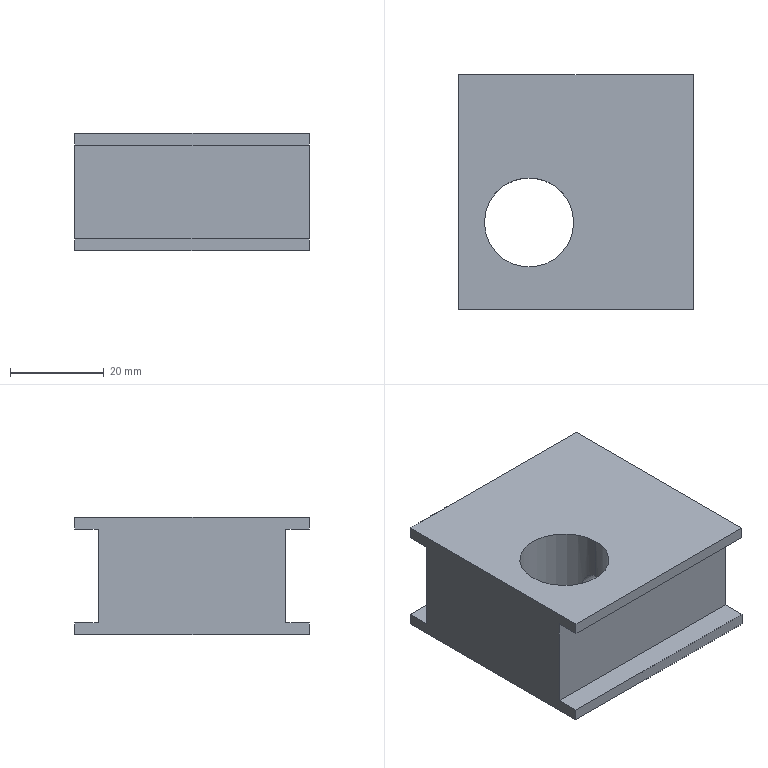Component | SolidWorks | TensionBlock-1 | 1 solid | 18 faces | box 50 x 50 x 25 mm | volume 44480 mm3 | plane 14 | cylinder 4 | commonest cylinder face diameters 6.8 x2 19 x2
build123d program:
from build123d import *

# Parameters (mm, degrees)
SKETCH1_W             = 50
SKETCH1_H             = 50
BOSS_EXTRUDE1_DEPTH   = 12.5
SKETCH2_W             = 20
SKETCH2_H             = 5
CUT_EXTRUDE1_DEPTH    = 58.282
SKETCH3_R             = 9.5
CUT_EXTRUDE2_DEPTH    = 25
M8_TAPPED_HOLE1_D     = 6.8
M8_TAPPED_HOLE1_DEPTH = 35
M8_TAPPED_HOLE1_TIP   = 2.043


with BuildPart() as part:
    # Sketch1 → Boss-Extrude1 (new, symmetric)
    with BuildSketch(Plane(origin=(0, 0, 0), x_dir=(0, 0, -1), z_dir=(1, 0, 0))):
        Rectangle(SKETCH1_W, SKETCH1_H)
    extrude(amount=BOSS_EXTRUDE1_DEPTH, both=True)

    # Sketch2 → Cut-Extrude1 (cut, through all)
    with BuildSketch(Plane(origin=(0, 0, -25), x_dir=(-1, 0, 0), z_dir=(0, 0, -1))):
        with Locations((0, 22.5)):
            Rectangle(SKETCH2_W, SKETCH2_H)
        with Locations((0, -22.5)):
            Rectangle(SKETCH2_W, SKETCH2_H)
    extrude(amount=-CUT_EXTRUDE1_DEPTH, mode=Mode.SUBTRACT)

    # Sketch3 → Cut-Extrude2 (cut)
    with BuildSketch(Plane(origin=(12.5, 0, 0), x_dir=(0, 0, -1), z_dir=(1, 0, 0))):
        with Locations((10, -6.5)):
            Circle(SKETCH3_R)
    extrude(amount=-CUT_EXTRUDE2_DEPTH, mode=Mode.SUBTRACT)

    # M8 Tapped Hole1
    with Locations(Plane.XY.offset(25)):
        with Locations((0, -6.5)):
            Hole(M8_TAPPED_HOLE1_D / 2, depth=M8_TAPPED_HOLE1_DEPTH)
            with Locations((0, 0, -(M8_TAPPED_HOLE1_DEPTH + M8_TAPPED_HOLE1_TIP / 2))):  # 118° drill point
                Cone(0, M8_TAPPED_HOLE1_D / 2, M8_TAPPED_HOLE1_TIP, mode=Mode.SUBTRACT)


solid = part.part

# Placed as in the assembly
solid = solid.moved(Location((235.493, -33.411, 631), (0, 90, 0)))
STEP:
#1=COLOUR_RGB('',0.7922,0.8196,0.9333);
#2=FILL_AREA_STYLE_COLOUR('',#1);
#3=FILL_AREA_STYLE('',(#2));
#4=SURFACE_STYLE_FILL_AREA(#3);
#5=SURFACE_SIDE_STYLE('',(#4));
#6=SURFACE_STYLE_USAGE(.BOTH.,#5);
#7=PRESENTATION_STYLE_ASSIGNMENT((#6));
#8=CARTESIAN_POINT('',(9.252,-1.571,24.976));
#9=VERTEX_POINT('',#8);
#10=CARTESIAN_POINT('',(9.252,-1.571,24.709));
#11=VERTEX_POINT('',#10);
#12=CARTESIAN_POINT('',(9.252,-1.571,24.976));
#13=CARTESIAN_POINT('',(9.252,-1.58,24.976));
#14=CARTESIAN_POINT('',(9.251,-1.589,24.976));
#15=CARTESIAN_POINT('',(9.25,-1.606,24.972));
#16=CARTESIAN_POINT('',(9.249,-1.615,24.969));
#17=CARTESIAN_POINT('',(9.247,-1.631,24.963));
#18=CARTESIAN_POINT('',(9.246,-1.639,24.959));
#19=CARTESIAN_POINT('',(9.243,-1.653,24.949));
#20=CARTESIAN_POINT('',(9.241,-1.66,24.943));
#21=CARTESIAN_POINT('',(9.238,-1.672,24.931));
#22=CARTESIAN_POINT('',(9.236,-1.678,24.924));
#23=CARTESIAN_POINT('',(9.233,-1.687,24.91));
#24=CARTESIAN_POINT('',(9.232,-1.692,24.902));
#25=CARTESIAN_POINT('',(9.23,-1.698,24.886));
#26=CARTESIAN_POINT('',(9.229,-1.701,24.877));
#27=CARTESIAN_POINT('',(9.227,-1.704,24.86));
#28=CARTESIAN_POINT('',(9.227,-1.705,24.851));
#29=CARTESIAN_POINT('',(9.227,-1.705,24.834));
#30=CARTESIAN_POINT('',(9.227,-1.704,24.825));
#31=CARTESIAN_POINT('',(9.229,-1.701,24.808));
#32=CARTESIAN_POINT('',(9.23,-1.698,24.799));
#33=CARTESIAN_POINT('',(9.232,-1.692,24.783));
#34=CARTESIAN_POINT('',(9.233,-1.687,24.775));
#35=CARTESIAN_POINT('',(9.236,-1.678,24.761));
#36=CARTESIAN_POINT('',(9.238,-1.672,24.754));
#37=CARTESIAN_POINT('',(9.241,-1.66,24.742));
#38=CARTESIAN_POINT('',(9.243,-1.653,24.736));
#39=CARTESIAN_POINT('',(9.246,-1.639,24.726));
#40=CARTESIAN_POINT('',(9.247,-1.631,24.722));
#41=CARTESIAN_POINT('',(9.249,-1.615,24.716));
#42=CARTESIAN_POINT('',(9.25,-1.606,24.713));
#43=CARTESIAN_POINT('',(9.251,-1.589,24.71));
#44=CARTESIAN_POINT('',(9.252,-1.58,24.709));
#45=CARTESIAN_POINT('',(9.252,-1.571,24.709));
#46=B_SPLINE_CURVE_WITH_KNOTS('',3,(#12,#13,#14,#15,#16,#17,#18,#19,#20,#21,#22,#23,#24,#25,#26,#27,#28,#29,#30,#31,#32,#33,#34,#35,#36,#37,#38,#39,#40,#41,#42,#43,#44,#45),.UNSPECIFIED.,.F.,.F.,(4,2,2,2,2,2,2,2,2,2,2,2,2,2,2,2,4),(0.01072,0.01139,0.01206,0.01273,0.0134,0.01407,0.01474,0.01541,0.01608,0.01675,0.01742,0.01809,0.01876,0.01943,0.0201,0.02077,0.02144),.UNSPECIFIED.);
#47=EDGE_CURVE('',#9,#11,#46,.T.);
#48=ORIENTED_EDGE('',*,*,#47,.F.);
#49=CARTESIAN_POINT('',(10.256,-1.571,24.976));
#50=VERTEX_POINT('',#49);
#51=CARTESIAN_POINT('',(10.256,-1.571,24.976));
#52=DIRECTION('',(1.,-0.,0.));
#53=VECTOR('',#52,39.37);
#54=LINE('',#51,#53);
#55=EDGE_CURVE('',#9,#50,#54,.T.);
#56=ORIENTED_EDGE('',*,*,#55,.T.);
#57=CARTESIAN_POINT('',(10.256,-1.571,24.709));
#58=VERTEX_POINT('',#57);
#59=CARTESIAN_POINT('',(10.256,-1.571,24.843));
#60=DIRECTION('',(1.,-0.,0.));
#61=DIRECTION('',(0.,0.,-1.));
#62=AXIS2_PLACEMENT_3D('',#59,#60,#61);
#63=CIRCLE('',#62,0.1339);
#64=EDGE_CURVE('',#50,#58,#63,.T.);
#65=ORIENTED_EDGE('',*,*,#64,.T.);
#66=CARTESIAN_POINT('',(10.256,-1.571,24.709));
#67=DIRECTION('',(1.,-0.,0.));
#68=VECTOR('',#67,39.37);
#69=LINE('',#66,#68);
#70=EDGE_CURVE('',#11,#58,#69,.T.);
#71=ORIENTED_EDGE('',*,*,#70,.F.);
#72=EDGE_LOOP('',(#48,#56,#65,#71));
#73=FACE_OUTER_BOUND('',#72,.T.);
#74=CARTESIAN_POINT('',(10.256,-1.571,24.843));
#75=DIRECTION('',(1.,-0.,0.));
#76=DIRECTION('',(0.,0.,-1.));
#77=AXIS2_PLACEMENT_3D('',#74,#75,#76);
#78=CYLINDRICAL_SURFACE('',#77,0.1339);
#79=ADVANCED_FACE('',(#73),#78,.F.);
#80=CARTESIAN_POINT('',(9.252,-1.571,25.335));
#81=VERTEX_POINT('',#80);
#82=CARTESIAN_POINT('',(8.504,-1.571,25.335));
#83=VERTEX_POINT('',#82);
#84=CARTESIAN_POINT('',(8.878,-1.571,25.335));
#85=DIRECTION('',(0.,0.,-1.));
#86=DIRECTION('',(-1.,0.,0.));
#87=AXIS2_PLACEMENT_3D('',#84,#85,#86);
#88=CIRCLE('',#87,0.374);
#89=EDGE_CURVE('',#81,#83,#88,.T.);
#90=ORIENTED_EDGE('',*,*,#89,.F.);
#91=CARTESIAN_POINT('',(9.252,-1.571,25.335));
#92=DIRECTION('',(0.,0.,-1.));
#93=VECTOR('',#92,39.37);
#94=LINE('',#91,#93);
#95=EDGE_CURVE('',#81,#9,#94,.T.);
#96=ORIENTED_EDGE('',*,*,#95,.T.);
#97=ORIENTED_EDGE('',*,*,#47,.T.);
#98=CARTESIAN_POINT('',(9.252,-1.571,24.35));
#99=VERTEX_POINT('',#98);
#100=CARTESIAN_POINT('',(9.252,-1.571,25.335));
#101=DIRECTION('',(0.,0.,-1.));
#102=VECTOR('',#101,39.37);
#103=LINE('',#100,#102);
#104=EDGE_CURVE('',#11,#99,#103,.T.);
#105=ORIENTED_EDGE('',*,*,#104,.T.);
#106=CARTESIAN_POINT('',(8.504,-1.571,24.35));
#107=VERTEX_POINT('',#106);
#108=CARTESIAN_POINT('',(8.878,-1.571,24.35));
#109=DIRECTION('',(0.,0.,-1.));
#110=DIRECTION('',(-1.,0.,0.));
#111=AXIS2_PLACEMENT_3D('',#108,#109,#110);
#112=CIRCLE('',#111,0.374);
#113=EDGE_CURVE('',#99,#107,#112,.T.);
#114=ORIENTED_EDGE('',*,*,#113,.T.);
#115=CARTESIAN_POINT('',(8.504,-1.571,25.335));
#116=DIRECTION('',(0.,0.,-1.));
#117=VECTOR('',#116,39.37);
#118=LINE('',#115,#117);
#119=EDGE_CURVE('',#83,#107,#118,.T.);
#120=ORIENTED_EDGE('',*,*,#119,.F.);
#121=EDGE_LOOP('',(#90,#96,#97,#105,#114,#120));
#122=FACE_OUTER_BOUND('',#121,.T.);
#123=CARTESIAN_POINT('',(8.878,-1.571,25.335));
#124=DIRECTION('',(0.,0.,-1.));
#125=DIRECTION('',(-1.,0.,0.));
#126=AXIS2_PLACEMENT_3D('',#123,#124,#125);
#127=CYLINDRICAL_SURFACE('',#126,0.374);
#128=ADVANCED_FACE('',(#122),#127,.F.);
#129=CARTESIAN_POINT('',(10.256,-2.3,24.35));
#130=VERTEX_POINT('',#129);
#131=CARTESIAN_POINT('',(10.256,-2.3,24.449));
#132=VERTEX_POINT('',#131);
#133=CARTESIAN_POINT('',(10.256,-2.3,24.35));
#134=DIRECTION('',(-0.,-0.,1.));
#135=VECTOR('',#134,39.37);
#136=LINE('',#133,#135);
#137=EDGE_CURVE('',#130,#132,#136,.T.);
#138=ORIENTED_EDGE('',*,*,#137,.T.);
#139=CARTESIAN_POINT('',(8.287,-2.3,24.449));
#140=VERTEX_POINT('',#139);
#141=CARTESIAN_POINT('',(10.256,-2.3,24.449));
#142=DIRECTION('',(-1.,0.,-0.));
#143=VECTOR('',#142,39.37);
#144=LINE('',#141,#143);
#145=EDGE_CURVE('',#132,#140,#144,.T.);
#146=ORIENTED_EDGE('',*,*,#145,.T.);
#147=CARTESIAN_POINT('',(8.287,-2.3,24.35));
#148=VERTEX_POINT('',#147);
#149=CARTESIAN_POINT('',(8.287,-2.3,24.35));
#150=DIRECTION('',(-0.,-0.,1.));
#151=VECTOR('',#150,39.37);
#152=LINE('',#149,#151);
#153=EDGE_CURVE('',#148,#140,#152,.T.);
#154=ORIENTED_EDGE('',*,*,#153,.F.);
#155=CARTESIAN_POINT('',(8.287,-2.3,24.35));
#156=DIRECTION('',(-1.,0.,-0.));
#157=VECTOR('',#156,39.37);
#158=LINE('',#155,#157);
#159=EDGE_CURVE('',#130,#148,#158,.T.);
#160=ORIENTED_EDGE('',*,*,#159,.F.);
#161=EDGE_LOOP('',(#138,#146,#154,#160));
#162=FACE_OUTER_BOUND('',#161,.T.);
#163=CARTESIAN_POINT('',(8.287,-2.3,24.35));
#164=DIRECTION('',(0.,1.,0.));
#165=DIRECTION('',(1.,-0.,0.));
#166=AXIS2_PLACEMENT_3D('',#163,#164,#165);
#167=PLANE('',#166);
#168=ADVANCED_FACE('',(#162),#167,.F.);
#169=CARTESIAN_POINT('',(8.287,-0.3312,24.35));
#170=VERTEX_POINT('',#169);
#171=CARTESIAN_POINT('',(8.287,-0.3312,24.449));
#172=VERTEX_POINT('',#171);
#173=CARTESIAN_POINT('',(8.287,-0.3312,24.35));
#174=DIRECTION('',(-0.,-0.,1.));
#175=VECTOR('',#174,39.37);
#176=LINE('',#173,#175);
#177=EDGE_CURVE('',#170,#172,#176,.T.);
#178=ORIENTED_EDGE('',*,*,#177,.T.);
#179=CARTESIAN_POINT('',(10.256,-0.3312,24.449));
#180=VERTEX_POINT('',#179);
#181=CARTESIAN_POINT('',(10.256,-0.3312,24.449));
#182=DIRECTION('',(-1.,0.,-0.));
#183=VECTOR('',#182,39.37);
#184=LINE('',#181,#183);
#185=EDGE_CURVE('',#180,#172,#184,.T.);
#186=ORIENTED_EDGE('',*,*,#185,.F.);
#187=CARTESIAN_POINT('',(10.256,-0.3312,24.35));
#188=VERTEX_POINT('',#187);
#189=CARTESIAN_POINT('',(10.256,-0.3312,24.35));
#190=DIRECTION('',(-0.,-0.,1.));
#191=VECTOR('',#190,39.37);
#192=LINE('',#189,#191);
#193=EDGE_CURVE('',#188,#180,#192,.T.);
#194=ORIENTED_EDGE('',*,*,#193,.F.);
#195=CARTESIAN_POINT('',(8.287,-0.3312,24.35));
#196=DIRECTION('',(1.,-0.,0.));
#197=VECTOR('',#196,39.37);
#198=LINE('',#195,#197);
#199=EDGE_CURVE('',#170,#188,#198,.T.);
#200=ORIENTED_EDGE('',*,*,#199,.F.);
#201=EDGE_LOOP('',(#178,#186,#194,#200));
#202=FACE_OUTER_BOUND('',#201,.T.);
#203=CARTESIAN_POINT('',(8.287,-0.3312,24.35));
#204=DIRECTION('',(-0.,-1.,-0.));
#205=DIRECTION('',(-1.,0.,-0.));
#206=AXIS2_PLACEMENT_3D('',#203,#204,#205);
#207=PLANE('',#206);
#208=ADVANCED_FACE('',(#202),#207,.F.);
#209=CARTESIAN_POINT('',(10.256,-1.571,24.843));
#210=DIRECTION('',(1.,-0.,0.));
#211=DIRECTION('',(0.,0.,-1.));
#212=AXIS2_PLACEMENT_3D('',#209,#210,#211);
#213=CIRCLE('',#212,0.1339);
#214=EDGE_CURVE('',#58,#50,#213,.T.);
#215=ORIENTED_EDGE('',*,*,#214,.F.);
#216=ORIENTED_EDGE('',*,*,#64,.F.);
#217=EDGE_LOOP('',(#215,#216));
#218=FACE_BOUND('',#217,.T.);
#219=CARTESIAN_POINT('',(10.256,-2.103,25.236));
#220=VERTEX_POINT('',#219);
#221=CARTESIAN_POINT('',(10.256,-2.103,24.449));
#222=VERTEX_POINT('',#221);
#223=CARTESIAN_POINT('',(10.256,-2.103,24.449));
#224=DIRECTION('',(0.,0.,-1.));
#225=VECTOR('',#224,39.37);
#226=LINE('',#223,#225);
#227=EDGE_CURVE('',#220,#222,#226,.T.);
#228=ORIENTED_EDGE('',*,*,#227,.T.);
#229=CARTESIAN_POINT('',(10.256,-2.3,24.449));
#230=DIRECTION('',(-0.,-1.,-0.));
#231=VECTOR('',#230,39.37);
#232=LINE('',#229,#231);
#233=EDGE_CURVE('',#222,#132,#232,.T.);
#234=ORIENTED_EDGE('',*,*,#233,.T.);
#235=ORIENTED_EDGE('',*,*,#137,.F.);
#236=CARTESIAN_POINT('',(10.256,-2.3,24.35));
#237=DIRECTION('',(-0.,-1.,-0.));
#238=VECTOR('',#237,39.37);
#239=LINE('',#236,#238);
#240=EDGE_CURVE('',#188,#130,#239,.T.);
#241=ORIENTED_EDGE('',*,*,#240,.F.);
#242=ORIENTED_EDGE('',*,*,#193,.T.);
#243=CARTESIAN_POINT('',(10.256,-0.528,24.449));
#244=VERTEX_POINT('',#243);
#245=CARTESIAN_POINT('',(10.256,-0.3312,24.449));
#246=DIRECTION('',(-0.,-1.,0.));
#247=VECTOR('',#246,39.37);
#248=LINE('',#245,#247);
#249=EDGE_CURVE('',#180,#244,#248,.T.);
#250=ORIENTED_EDGE('',*,*,#249,.T.);
#251=CARTESIAN_POINT('',(10.256,-0.528,25.236));
#252=VERTEX_POINT('',#251);
#253=CARTESIAN_POINT('',(10.256,-0.528,24.449));
#254=DIRECTION('',(-0.,-0.,1.));
#255=VECTOR('',#254,39.37);
#256=LINE('',#253,#255);
#257=EDGE_CURVE('',#244,#252,#256,.T.);
#258=ORIENTED_EDGE('',*,*,#257,.T.);
#259=CARTESIAN_POINT('',(10.256,-0.3312,25.236));
#260=VERTEX_POINT('',#259);
#261=CARTESIAN_POINT('',(10.256,-0.3312,25.236));
#262=DIRECTION('',(0.,1.,0.));
#263=VECTOR('',#262,39.37);
#264=LINE('',#261,#263);
#265=EDGE_CURVE('',#252,#260,#264,.T.);
#266=ORIENTED_EDGE('',*,*,#265,.T.);
#267=CARTESIAN_POINT('',(10.256,-0.3312,25.335));
#268=VERTEX_POINT('',#267);
#269=CARTESIAN_POINT('',(10.256,-0.3312,24.35));
#270=DIRECTION('',(-0.,-0.,1.));
#271=VECTOR('',#270,39.37);
#272=LINE('',#269,#271);
#273=EDGE_CURVE('',#260,#268,#272,.T.);
#274=ORIENTED_EDGE('',*,*,#273,.T.);
#275=CARTESIAN_POINT('',(10.256,-2.3,25.335));
#276=VERTEX_POINT('',#275);
#277=CARTESIAN_POINT('',(10.256,-2.3,25.335));
#278=DIRECTION('',(-0.,-1.,-0.));
#279=VECTOR('',#278,39.37);
#280=LINE('',#277,#279);
#281=EDGE_CURVE('',#268,#276,#280,.T.);
#282=ORIENTED_EDGE('',*,*,#281,.T.);
#283=CARTESIAN_POINT('',(10.256,-2.3,25.236));
#284=VERTEX_POINT('',#283);
#285=CARTESIAN_POINT('',(10.256,-2.3,24.35));
#286=DIRECTION('',(-0.,-0.,1.));
#287=VECTOR('',#286,39.37);
#288=LINE('',#285,#287);
#289=EDGE_CURVE('',#284,#276,#288,.T.);
#290=ORIENTED_EDGE('',*,*,#289,.F.);
#291=CARTESIAN_POINT('',(10.256,-2.3,25.236));
#292=DIRECTION('',(0.,1.,0.));
#293=VECTOR('',#292,39.37);
#294=LINE('',#291,#293);
#295=EDGE_CURVE('',#284,#220,#294,.T.);
#296=ORIENTED_EDGE('',*,*,#295,.T.);
#297=EDGE_LOOP('',(#228,#234,#235,#241,#242,#250,#258,#266,#274,#282,#290,#296));
#298=FACE_OUTER_BOUND('',#297,.T.);
#299=CARTESIAN_POINT('',(10.256,-2.3,24.35));
#300=DIRECTION('',(-1.,0.,-0.));
#301=DIRECTION('',(-0.,-0.,1.));
#302=AXIS2_PLACEMENT_3D('',#299,#300,#301);
#303=PLANE('',#302);
#304=ADVANCED_FACE('',(#218,#298),#303,.F.);
#305=CARTESIAN_POINT('',(8.287,-2.3,25.236));
#306=VERTEX_POINT('',#305);
#307=CARTESIAN_POINT('',(8.287,-2.3,25.335));
#308=VERTEX_POINT('',#307);
#309=CARTESIAN_POINT('',(8.287,-2.3,24.35));
#310=DIRECTION('',(-0.,-0.,1.));
#311=VECTOR('',#310,39.37);
#312=LINE('',#309,#311);
#313=EDGE_CURVE('',#306,#308,#312,.T.);
#314=ORIENTED_EDGE('',*,*,#313,.F.);
#315=CARTESIAN_POINT('',(10.256,-2.3,25.236));
#316=DIRECTION('',(-1.,0.,-0.));
#317=VECTOR('',#316,39.37);
#318=LINE('',#315,#317);
#319=EDGE_CURVE('',#284,#306,#318,.T.);
#320=ORIENTED_EDGE('',*,*,#319,.F.);
#321=ORIENTED_EDGE('',*,*,#289,.T.);
#322=CARTESIAN_POINT('',(8.287,-2.3,25.335));
#323=DIRECTION('',(-1.,0.,-0.));
#324=VECTOR('',#323,39.37);
#325=LINE('',#322,#324);
#326=EDGE_CURVE('',#276,#308,#325,.T.);
#327=ORIENTED_EDGE('',*,*,#326,.T.);
#328=EDGE_LOOP('',(#314,#320,#321,#327));
#329=FACE_OUTER_BOUND('',#328,.T.);
#330=CARTESIAN_POINT('',(8.287,-2.3,24.35));
#331=DIRECTION('',(0.,1.,0.));
#332=DIRECTION('',(1.,-0.,0.));
#333=AXIS2_PLACEMENT_3D('',#330,#331,#332);
#334=PLANE('',#333);
#335=ADVANCED_FACE('',(#329),#334,.F.);
#336=ORIENTED_EDGE('',*,*,#153,.T.);
#337=CARTESIAN_POINT('',(8.287,-2.103,24.449));
#338=VERTEX_POINT('',#337);
#339=CARTESIAN_POINT('',(8.287,-2.3,24.449));
#340=DIRECTION('',(-0.,-1.,-0.));
#341=VECTOR('',#340,39.37);
#342=LINE('',#339,#341);
#343=EDGE_CURVE('',#338,#140,#342,.T.);
#344=ORIENTED_EDGE('',*,*,#343,.F.);
#345=CARTESIAN_POINT('',(8.287,-2.103,25.236));
#346=VERTEX_POINT('',#345);
#347=CARTESIAN_POINT('',(8.287,-2.103,24.449));
#348=DIRECTION('',(0.,0.,-1.));
#349=VECTOR('',#348,39.37);
#350=LINE('',#347,#349);
#351=EDGE_CURVE('',#346,#338,#350,.T.);
#352=ORIENTED_EDGE('',*,*,#351,.F.);
#353=CARTESIAN_POINT('',(8.287,-2.3,25.236));
#354=DIRECTION('',(0.,1.,0.));
#355=VECTOR('',#354,39.37);
#356=LINE('',#353,#355);
#357=EDGE_CURVE('',#306,#346,#356,.T.);
#358=ORIENTED_EDGE('',*,*,#357,.F.);
#359=ORIENTED_EDGE('',*,*,#313,.T.);
#360=CARTESIAN_POINT('',(8.287,-0.3312,25.335));
#361=VERTEX_POINT('',#360);
#362=CARTESIAN_POINT('',(8.287,-2.3,25.335));
#363=DIRECTION('',(0.,1.,0.));
#364=VECTOR('',#363,39.37);
#365=LINE('',#362,#364);
#366=EDGE_CURVE('',#308,#361,#365,.T.);
#367=ORIENTED_EDGE('',*,*,#366,.T.);
#368=CARTESIAN_POINT('',(8.287,-0.3312,25.236));
#369=VERTEX_POINT('',#368);
#370=CARTESIAN_POINT('',(8.287,-0.3312,24.35));
#371=DIRECTION('',(-0.,-0.,1.));
#372=VECTOR('',#371,39.37);
#373=LINE('',#370,#372);
#374=EDGE_CURVE('',#369,#361,#373,.T.);
#375=ORIENTED_EDGE('',*,*,#374,.F.);
#376=CARTESIAN_POINT('',(8.287,-0.528,25.236));
#377=VERTEX_POINT('',#376);
#378=CARTESIAN_POINT('',(8.287,-0.3312,25.236));
#379=DIRECTION('',(0.,1.,0.));
#380=VECTOR('',#379,39.37);
#381=LINE('',#378,#380);
#382=EDGE_CURVE('',#377,#369,#381,.T.);
#383=ORIENTED_EDGE('',*,*,#382,.F.);
#384=CARTESIAN_POINT('',(8.287,-0.528,24.449));
#385=VERTEX_POINT('',#384);
#386=CARTESIAN_POINT('',(8.287,-0.528,24.449));
#387=DIRECTION('',(-0.,-0.,1.));
#388=VECTOR('',#387,39.37);
#389=LINE('',#386,#388);
#390=EDGE_CURVE('',#385,#377,#389,.T.);
#391=ORIENTED_EDGE('',*,*,#390,.F.);
#392=CARTESIAN_POINT('',(8.287,-0.3312,24.449));
#393=DIRECTION('',(-0.,-1.,0.));
#394=VECTOR('',#393,39.37);
#395=LINE('',#392,#394);
#396=EDGE_CURVE('',#172,#385,#395,.T.);
#397=ORIENTED_EDGE('',*,*,#396,.F.);
#398=ORIENTED_EDGE('',*,*,#177,.F.);
#399=CARTESIAN_POINT('',(8.287,-2.3,24.35));
#400=DIRECTION('',(0.,1.,0.));
#401=VECTOR('',#400,39.37);
#402=LINE('',#399,#401);
#403=EDGE_CURVE('',#148,#170,#402,.T.);
#404=ORIENTED_EDGE('',*,*,#403,.F.);
#405=EDGE_LOOP('',(#336,#344,#352,#358,#359,#367,#375,#383,#391,#397,#398,#404));
#406=FACE_OUTER_BOUND('',#405,.T.);
#407=CARTESIAN_POINT('',(8.287,-2.3,24.35));
#408=DIRECTION('',(1.,-0.,0.));
#409=DIRECTION('',(0.,0.,-1.));
#410=AXIS2_PLACEMENT_3D('',#407,#408,#409);
#411=PLANE('',#410);
#412=ADVANCED_FACE('',(#406),#411,.F.);
#413=ORIENTED_EDGE('',*,*,#273,.F.);
#414=CARTESIAN_POINT('',(10.256,-0.3312,25.236));
#415=DIRECTION('',(-1.,0.,-0.));
#416=VECTOR('',#415,39.37);
#417=LINE('',#414,#416);
#418=EDGE_CURVE('',#260,#369,#417,.T.);
#419=ORIENTED_EDGE('',*,*,#418,.T.);
#420=ORIENTED_EDGE('',*,*,#374,.T.);
#421=CARTESIAN_POINT('',(8.287,-0.3312,25.335));
#422=DIRECTION('',(1.,-0.,0.));
#423=VECTOR('',#422,39.37);
#424=LINE('',#421,#423);
#425=EDGE_CURVE('',#361,#268,#424,.T.);
#426=ORIENTED_EDGE('',*,*,#425,.T.);
#427=EDGE_LOOP('',(#413,#419,#420,#426));
#428=FACE_OUTER_BOUND('',#427,.T.);
#429=CARTESIAN_POINT('',(8.287,-0.3312,24.35));
#430=DIRECTION('',(-0.,-1.,-0.));
#431=DIRECTION('',(-1.,0.,-0.));
#432=AXIS2_PLACEMENT_3D('',#429,#430,#431);
#433=PLANE('',#432);
#434=ADVANCED_FACE('',(#428),#433,.F.);
#435=CARTESIAN_POINT('',(8.878,-1.571,24.35));
#436=DIRECTION('',(0.,0.,-1.));
#437=DIRECTION('',(-1.,0.,0.));
#438=AXIS2_PLACEMENT_3D('',#435,#436,#437);
#439=CIRCLE('',#438,0.374);
#440=EDGE_CURVE('',#107,#99,#439,.T.);
#441=ORIENTED_EDGE('',*,*,#440,.F.);
#442=ORIENTED_EDGE('',*,*,#113,.F.);
#443=EDGE_LOOP('',(#441,#442));
#444=FACE_BOUND('',#443,.T.);
#445=ORIENTED_EDGE('',*,*,#240,.T.);
#446=ORIENTED_EDGE('',*,*,#159,.T.);
#447=ORIENTED_EDGE('',*,*,#403,.T.);
#448=ORIENTED_EDGE('',*,*,#199,.T.);
#449=EDGE_LOOP('',(#445,#446,#447,#448));
#450=FACE_OUTER_BOUND('',#449,.T.);
#451=CARTESIAN_POINT('',(9.271,-1.315,24.35));
#452=DIRECTION('',(0.,0.,-1.));
#453=DIRECTION('',(-1.,0.,-0.));
#454=AXIS2_PLACEMENT_3D('',#451,#452,#453);
#455=PLANE('',#454);
#456=ADVANCED_FACE('',(#444,#450),#455,.T.);
#457=CARTESIAN_POINT('',(8.878,-1.571,25.335));
#458=DIRECTION('',(0.,0.,-1.));
#459=DIRECTION('',(-1.,0.,0.));
#460=AXIS2_PLACEMENT_3D('',#457,#458,#459);
#461=CIRCLE('',#460,0.374);
#462=EDGE_CURVE('',#83,#81,#461,.T.);
#463=ORIENTED_EDGE('',*,*,#462,.T.);
#464=ORIENTED_EDGE('',*,*,#89,.T.);
#465=EDGE_LOOP('',(#463,#464));
#466=FACE_BOUND('',#465,.T.);
#467=ORIENTED_EDGE('',*,*,#281,.F.);
#468=ORIENTED_EDGE('',*,*,#425,.F.);
#469=ORIENTED_EDGE('',*,*,#366,.F.);
#470=ORIENTED_EDGE('',*,*,#326,.F.);
#471=EDGE_LOOP('',(#467,#468,#469,#470));
#472=FACE_OUTER_BOUND('',#471,.T.);
#473=CARTESIAN_POINT('',(9.271,-1.315,25.335));
#474=DIRECTION('',(0.,0.,-1.));
#475=DIRECTION('',(-1.,0.,-0.));
#476=AXIS2_PLACEMENT_3D('',#473,#474,#475);
#477=PLANE('',#476);
#478=ADVANCED_FACE('',(#466,#472),#477,.F.);
#479=ORIENTED_EDGE('',*,*,#396,.T.);
#480=CARTESIAN_POINT('',(10.256,-0.528,24.449));
#481=DIRECTION('',(-1.,0.,-0.));
#482=VECTOR('',#481,39.37);
#483=LINE('',#480,#482);
#484=EDGE_CURVE('',#244,#385,#483,.T.);
#485=ORIENTED_EDGE('',*,*,#484,.F.);
#486=ORIENTED_EDGE('',*,*,#249,.F.);
#487=ORIENTED_EDGE('',*,*,#185,.T.);
#488=EDGE_LOOP('',(#479,#485,#486,#487));
#489=FACE_OUTER_BOUND('',#488,.T.);
#490=CARTESIAN_POINT('',(10.256,-0.3312,24.449));
#491=DIRECTION('',(0.,-0.,-1.));
#492=DIRECTION('',(0.,1.,-0.));
#493=AXIS2_PLACEMENT_3D('',#490,#491,#492);
#494=PLANE('',#493);
#495=ADVANCED_FACE('',(#489),#494,.F.);
#496=ORIENTED_EDGE('',*,*,#382,.T.);
#497=ORIENTED_EDGE('',*,*,#418,.F.);
#498=ORIENTED_EDGE('',*,*,#265,.F.);
#499=CARTESIAN_POINT('',(10.256,-0.528,25.236));
#500=DIRECTION('',(-1.,0.,-0.));
#501=VECTOR('',#500,39.37);
#502=LINE('',#499,#501);
#503=EDGE_CURVE('',#252,#377,#502,.T.);
#504=ORIENTED_EDGE('',*,*,#503,.T.);
#505=EDGE_LOOP('',(#496,#497,#498,#504));
#506=FACE_OUTER_BOUND('',#505,.T.);
#507=CARTESIAN_POINT('',(10.256,-0.3312,25.236));
#508=DIRECTION('',(-0.,-0.,1.));
#509=DIRECTION('',(1.,-0.,0.));
#510=AXIS2_PLACEMENT_3D('',#507,#508,#509);
#511=PLANE('',#510);
#512=ADVANCED_FACE('',(#506),#511,.F.);
#513=ORIENTED_EDGE('',*,*,#390,.T.);
#514=ORIENTED_EDGE('',*,*,#503,.F.);
#515=ORIENTED_EDGE('',*,*,#257,.F.);
#516=ORIENTED_EDGE('',*,*,#484,.T.);
#517=EDGE_LOOP('',(#513,#514,#515,#516));
#518=FACE_OUTER_BOUND('',#517,.T.);
#519=CARTESIAN_POINT('',(10.256,-0.528,24.449));
#520=DIRECTION('',(-0.,-1.,-0.));
#521=DIRECTION('',(-1.,0.,-0.));
#522=AXIS2_PLACEMENT_3D('',#519,#520,#521);
#523=PLANE('',#522);
#524=ADVANCED_FACE('',(#518),#523,.F.);
#525=ORIENTED_EDGE('',*,*,#343,.T.);
#526=ORIENTED_EDGE('',*,*,#145,.F.);
#527=ORIENTED_EDGE('',*,*,#233,.F.);
#528=CARTESIAN_POINT('',(10.256,-2.103,24.449));
#529=DIRECTION('',(-1.,0.,-0.));
#530=VECTOR('',#529,39.37);
#531=LINE('',#528,#530);
#532=EDGE_CURVE('',#222,#338,#531,.T.);
#533=ORIENTED_EDGE('',*,*,#532,.T.);
#534=EDGE_LOOP('',(#525,#526,#527,#533));
#535=FACE_OUTER_BOUND('',#534,.T.);
#536=CARTESIAN_POINT('',(10.256,-2.3,24.449));
#537=DIRECTION('',(0.,0.,-1.));
#538=DIRECTION('',(-1.,0.,-0.));
#539=AXIS2_PLACEMENT_3D('',#536,#537,#538);
#540=PLANE('',#539);
#541=ADVANCED_FACE('',(#535),#540,.F.);
#542=ORIENTED_EDGE('',*,*,#351,.T.);
#543=ORIENTED_EDGE('',*,*,#532,.F.);
#544=ORIENTED_EDGE('',*,*,#227,.F.);
#545=CARTESIAN_POINT('',(10.256,-2.103,25.236));
#546=DIRECTION('',(-1.,0.,-0.));
#547=VECTOR('',#546,39.37);
#548=LINE('',#545,#547);
#549=EDGE_CURVE('',#220,#346,#548,.T.);
#550=ORIENTED_EDGE('',*,*,#549,.T.);
#551=EDGE_LOOP('',(#542,#543,#544,#550));
#552=FACE_OUTER_BOUND('',#551,.T.);
#553=CARTESIAN_POINT('',(10.256,-2.103,24.449));
#554=DIRECTION('',(0.,1.,0.));
#555=DIRECTION('',(1.,-0.,0.));
#556=AXIS2_PLACEMENT_3D('',#553,#554,#555);
#557=PLANE('',#556);
#558=ADVANCED_FACE('',(#552),#557,.F.);
#559=ORIENTED_EDGE('',*,*,#357,.T.);
#560=ORIENTED_EDGE('',*,*,#549,.F.);
#561=ORIENTED_EDGE('',*,*,#295,.F.);
#562=ORIENTED_EDGE('',*,*,#319,.T.);
#563=EDGE_LOOP('',(#559,#560,#561,#562));
#564=FACE_OUTER_BOUND('',#563,.T.);
#565=CARTESIAN_POINT('',(10.256,-2.3,25.236));
#566=DIRECTION('',(-0.,-0.,1.));
#567=DIRECTION('',(1.,-0.,0.));
#568=AXIS2_PLACEMENT_3D('',#565,#566,#567);
#569=PLANE('',#568);
#570=ADVANCED_FACE('',(#564),#569,.F.);
#571=ORIENTED_EDGE('',*,*,#95,.F.);
#572=ORIENTED_EDGE('',*,*,#462,.F.);
#573=ORIENTED_EDGE('',*,*,#119,.T.);
#574=ORIENTED_EDGE('',*,*,#440,.T.);
#575=ORIENTED_EDGE('',*,*,#104,.F.);
#576=CARTESIAN_POINT('',(9.252,-1.571,24.709));
#577=CARTESIAN_POINT('',(9.252,-1.562,24.709));
#578=CARTESIAN_POINT('',(9.251,-1.554,24.71));
#579=CARTESIAN_POINT('',(9.25,-1.536,24.713));
#580=CARTESIAN_POINT('',(9.249,-1.528,24.716));
#581=CARTESIAN_POINT('',(9.247,-1.512,24.722));
#582=CARTESIAN_POINT('',(9.246,-1.504,24.726));
#583=CARTESIAN_POINT('',(9.243,-1.49,24.736));
#584=CARTESIAN_POINT('',(9.241,-1.483,24.742));
#585=CARTESIAN_POINT('',(9.236,-1.464,24.76));
#586=CARTESIAN_POINT('',(9.233,-1.454,24.775));
#587=CARTESIAN_POINT('',(9.23,-1.444,24.799));
#588=CARTESIAN_POINT('',(9.229,-1.442,24.808));
#589=CARTESIAN_POINT('',(9.227,-1.438,24.825));
#590=CARTESIAN_POINT('',(9.227,-1.437,24.834));
#591=CARTESIAN_POINT('',(9.227,-1.437,24.851));
#592=CARTESIAN_POINT('',(9.227,-1.438,24.86));
#593=CARTESIAN_POINT('',(9.229,-1.442,24.877));
#594=CARTESIAN_POINT('',(9.23,-1.444,24.886));
#595=CARTESIAN_POINT('',(9.232,-1.451,24.902));
#596=CARTESIAN_POINT('',(9.233,-1.455,24.91));
#597=CARTESIAN_POINT('',(9.236,-1.465,24.924));
#598=CARTESIAN_POINT('',(9.238,-1.471,24.931));
#599=CARTESIAN_POINT('',(9.241,-1.483,24.943));
#600=CARTESIAN_POINT('',(9.243,-1.49,24.949));
#601=CARTESIAN_POINT('',(9.246,-1.504,24.959));
#602=CARTESIAN_POINT('',(9.247,-1.512,24.963));
#603=CARTESIAN_POINT('',(9.249,-1.528,24.969));
#604=CARTESIAN_POINT('',(9.25,-1.536,24.972));
#605=CARTESIAN_POINT('',(9.251,-1.554,24.976));
#606=CARTESIAN_POINT('',(9.252,-1.563,24.976));
#607=CARTESIAN_POINT('',(9.252,-1.571,24.976));
#608=B_SPLINE_CURVE_WITH_KNOTS('',3,(#576,#577,#578,#579,#580,#581,#582,#583,#584,#585,#586,#587,#588,#589,#590,#591,#592,#593,#594,#595,#596,#597,#598,#599,#600,#601,#602,#603,#604,#605,#606,#607),.UNSPECIFIED.,.F.,.F.,(4,2,2,2,2,2,2,2,2,2,2,2,2,2,2,4),(0.,0.00067,0.00134,0.00201,0.00268,0.00402,0.00469,0.00536,0.00603,0.0067,0.00737,0.00804,0.00871,0.00938,0.01005,0.01072),.UNSPECIFIED.);
#609=EDGE_CURVE('',#11,#9,#608,.T.);
#610=ORIENTED_EDGE('',*,*,#609,.T.);
#611=EDGE_LOOP('',(#571,#572,#573,#574,#575,#610));
#612=FACE_OUTER_BOUND('',#611,.T.);
#613=CARTESIAN_POINT('',(8.878,-1.571,25.335));
#614=DIRECTION('',(0.,0.,-1.));
#615=DIRECTION('',(-1.,0.,0.));
#616=AXIS2_PLACEMENT_3D('',#613,#614,#615);
#617=CYLINDRICAL_SURFACE('',#616,0.374);
#618=ADVANCED_FACE('',(#612),#617,.F.);
#619=ORIENTED_EDGE('',*,*,#55,.F.);
#620=ORIENTED_EDGE('',*,*,#609,.F.);
#621=ORIENTED_EDGE('',*,*,#70,.T.);
#622=ORIENTED_EDGE('',*,*,#214,.T.);
#623=EDGE_LOOP('',(#619,#620,#621,#622));
#624=FACE_OUTER_BOUND('',#623,.T.);
#625=CARTESIAN_POINT('',(10.256,-1.571,24.843));
#626=DIRECTION('',(1.,-0.,0.));
#627=DIRECTION('',(0.,0.,-1.));
#628=AXIS2_PLACEMENT_3D('',#625,#626,#627);
#629=CYLINDRICAL_SURFACE('',#628,0.1339);
#630=ADVANCED_FACE('',(#624),#629,.F.);
#631=CLOSED_SHELL('',(#79,#128,#168,#208,#304,#335,#412,#434,#456,#478,#495,#512,#524,#541,#558,#570,#618,#630));
#632=MANIFOLD_SOLID_BREP('',#631);
#633=STYLED_ITEM('',(#7),#632);
#634=(LENGTH_UNIT()NAMED_UNIT(*)SI_UNIT($,.METRE.));
#635=LENGTH_MEASURE_WITH_UNIT(LENGTH_MEASURE(0.0254),#634);
#636=DIMENSIONAL_EXPONENTS(1.,0.,0.,0.,0.,0.,0.);
#637=(CONVERSION_BASED_UNIT('',#635)LENGTH_UNIT()NAMED_UNIT(#636));
#638=UNCERTAINTY_MEASURE_WITH_UNIT(LENGTH_MEASURE(0.00001),#637,'','');
#639=(NAMED_UNIT(*)PLANE_ANGLE_UNIT()SI_UNIT($,.RADIAN.));
#640=(NAMED_UNIT(*)SI_UNIT($,.STERADIAN.)SOLID_ANGLE_UNIT());
#641=(GEOMETRIC_REPRESENTATION_CONTEXT(3)GLOBAL_UNCERTAINTY_ASSIGNED_CONTEXT((#638))GLOBAL_UNIT_ASSIGNED_CONTEXT((#637,#639,#640))REPRESENTATION_CONTEXT('',''));
#642=MECHANICAL_DESIGN_GEOMETRIC_PRESENTATION_REPRESENTATION('',(#633),#641);
#643=CARTESIAN_POINT('',(0.,0.,0.));
#644=DIRECTION('',(0.,0.,1.));
#645=DIRECTION('',(1.,0.,0.));
#646=AXIS2_PLACEMENT_3D('',#643,#644,#645);
#647=(LENGTH_UNIT()NAMED_UNIT(*)SI_UNIT($,.METRE.));
#648=LENGTH_MEASURE_WITH_UNIT(LENGTH_MEASURE(0.0254),#647);
#649=DIMENSIONAL_EXPONENTS(1.,0.,0.,0.,0.,0.,0.);
#650=(CONVERSION_BASED_UNIT('',#648)LENGTH_UNIT()NAMED_UNIT(#649));
#651=UNCERTAINTY_MEASURE_WITH_UNIT(LENGTH_MEASURE(0.00001),#650,'','');
#652=(NAMED_UNIT(*)PLANE_ANGLE_UNIT()SI_UNIT($,.RADIAN.));
#653=(NAMED_UNIT(*)SI_UNIT($,.STERADIAN.)SOLID_ANGLE_UNIT());
#654=(GEOMETRIC_REPRESENTATION_CONTEXT(3)GLOBAL_UNCERTAINTY_ASSIGNED_CONTEXT((#651))GLOBAL_UNIT_ASSIGNED_CONTEXT((#650,#652,#653))REPRESENTATION_CONTEXT('',''));
#655=ADVANCED_BREP_SHAPE_REPRESENTATION('',(#632,#646),#654);
#656=PRESENTATION_LAYER_ASSIGNMENT('','',(#633));